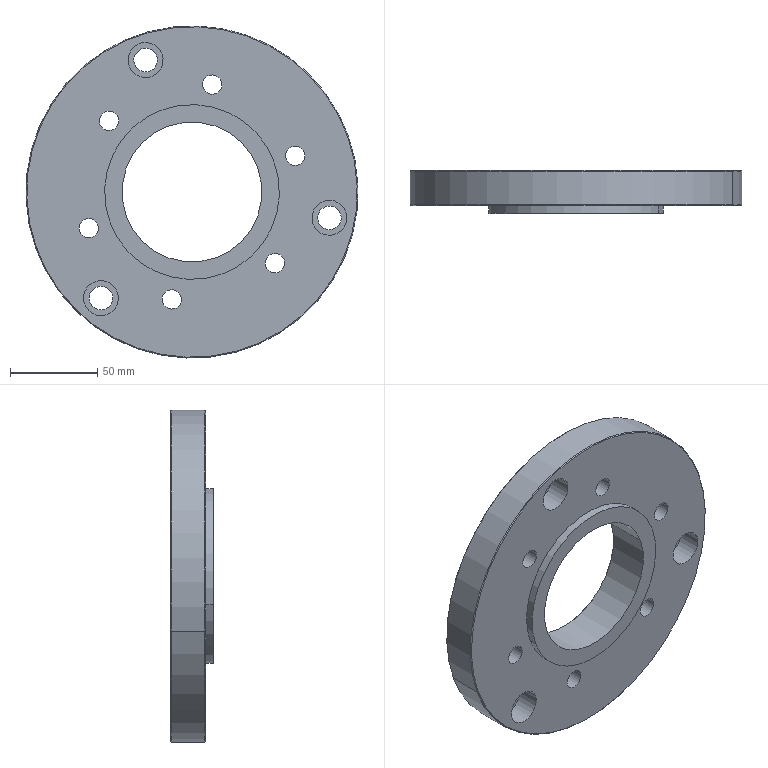Component | SolidWorks | 002AS-20130718-1_010A-20130717-1 | 1 solid | 60 faces | volume 441885 mm3 | cylinder 42 | plane 12 | cone 6 | commonest cylinder face diameters 18 x12 11 x12 20 x6 13.5 x6 100 x2 80 x2 190 x2